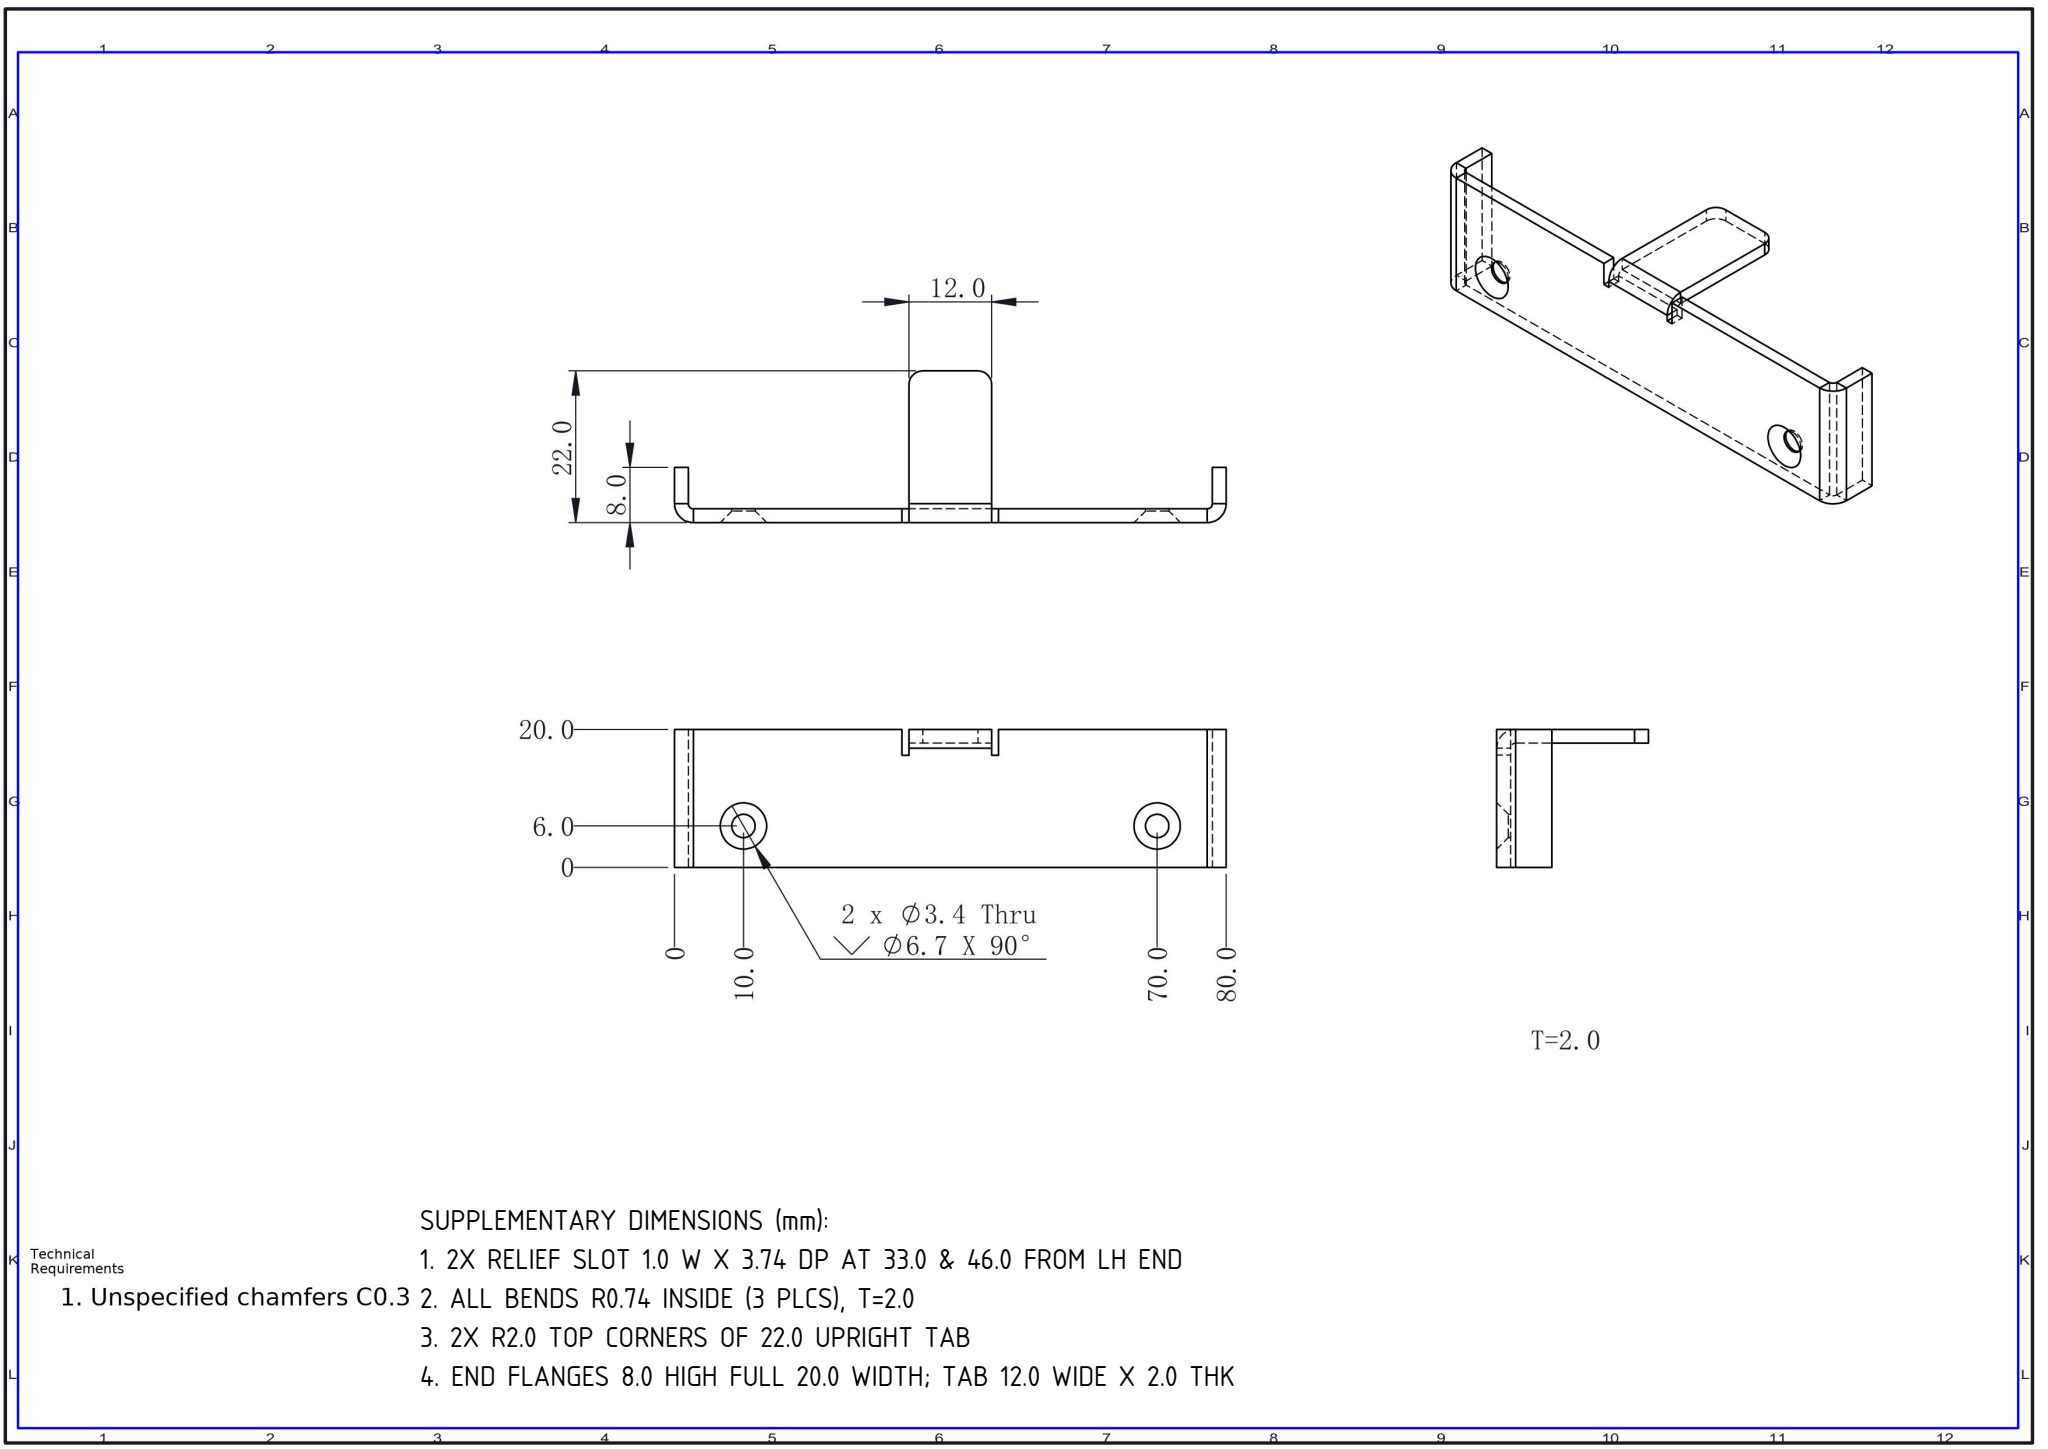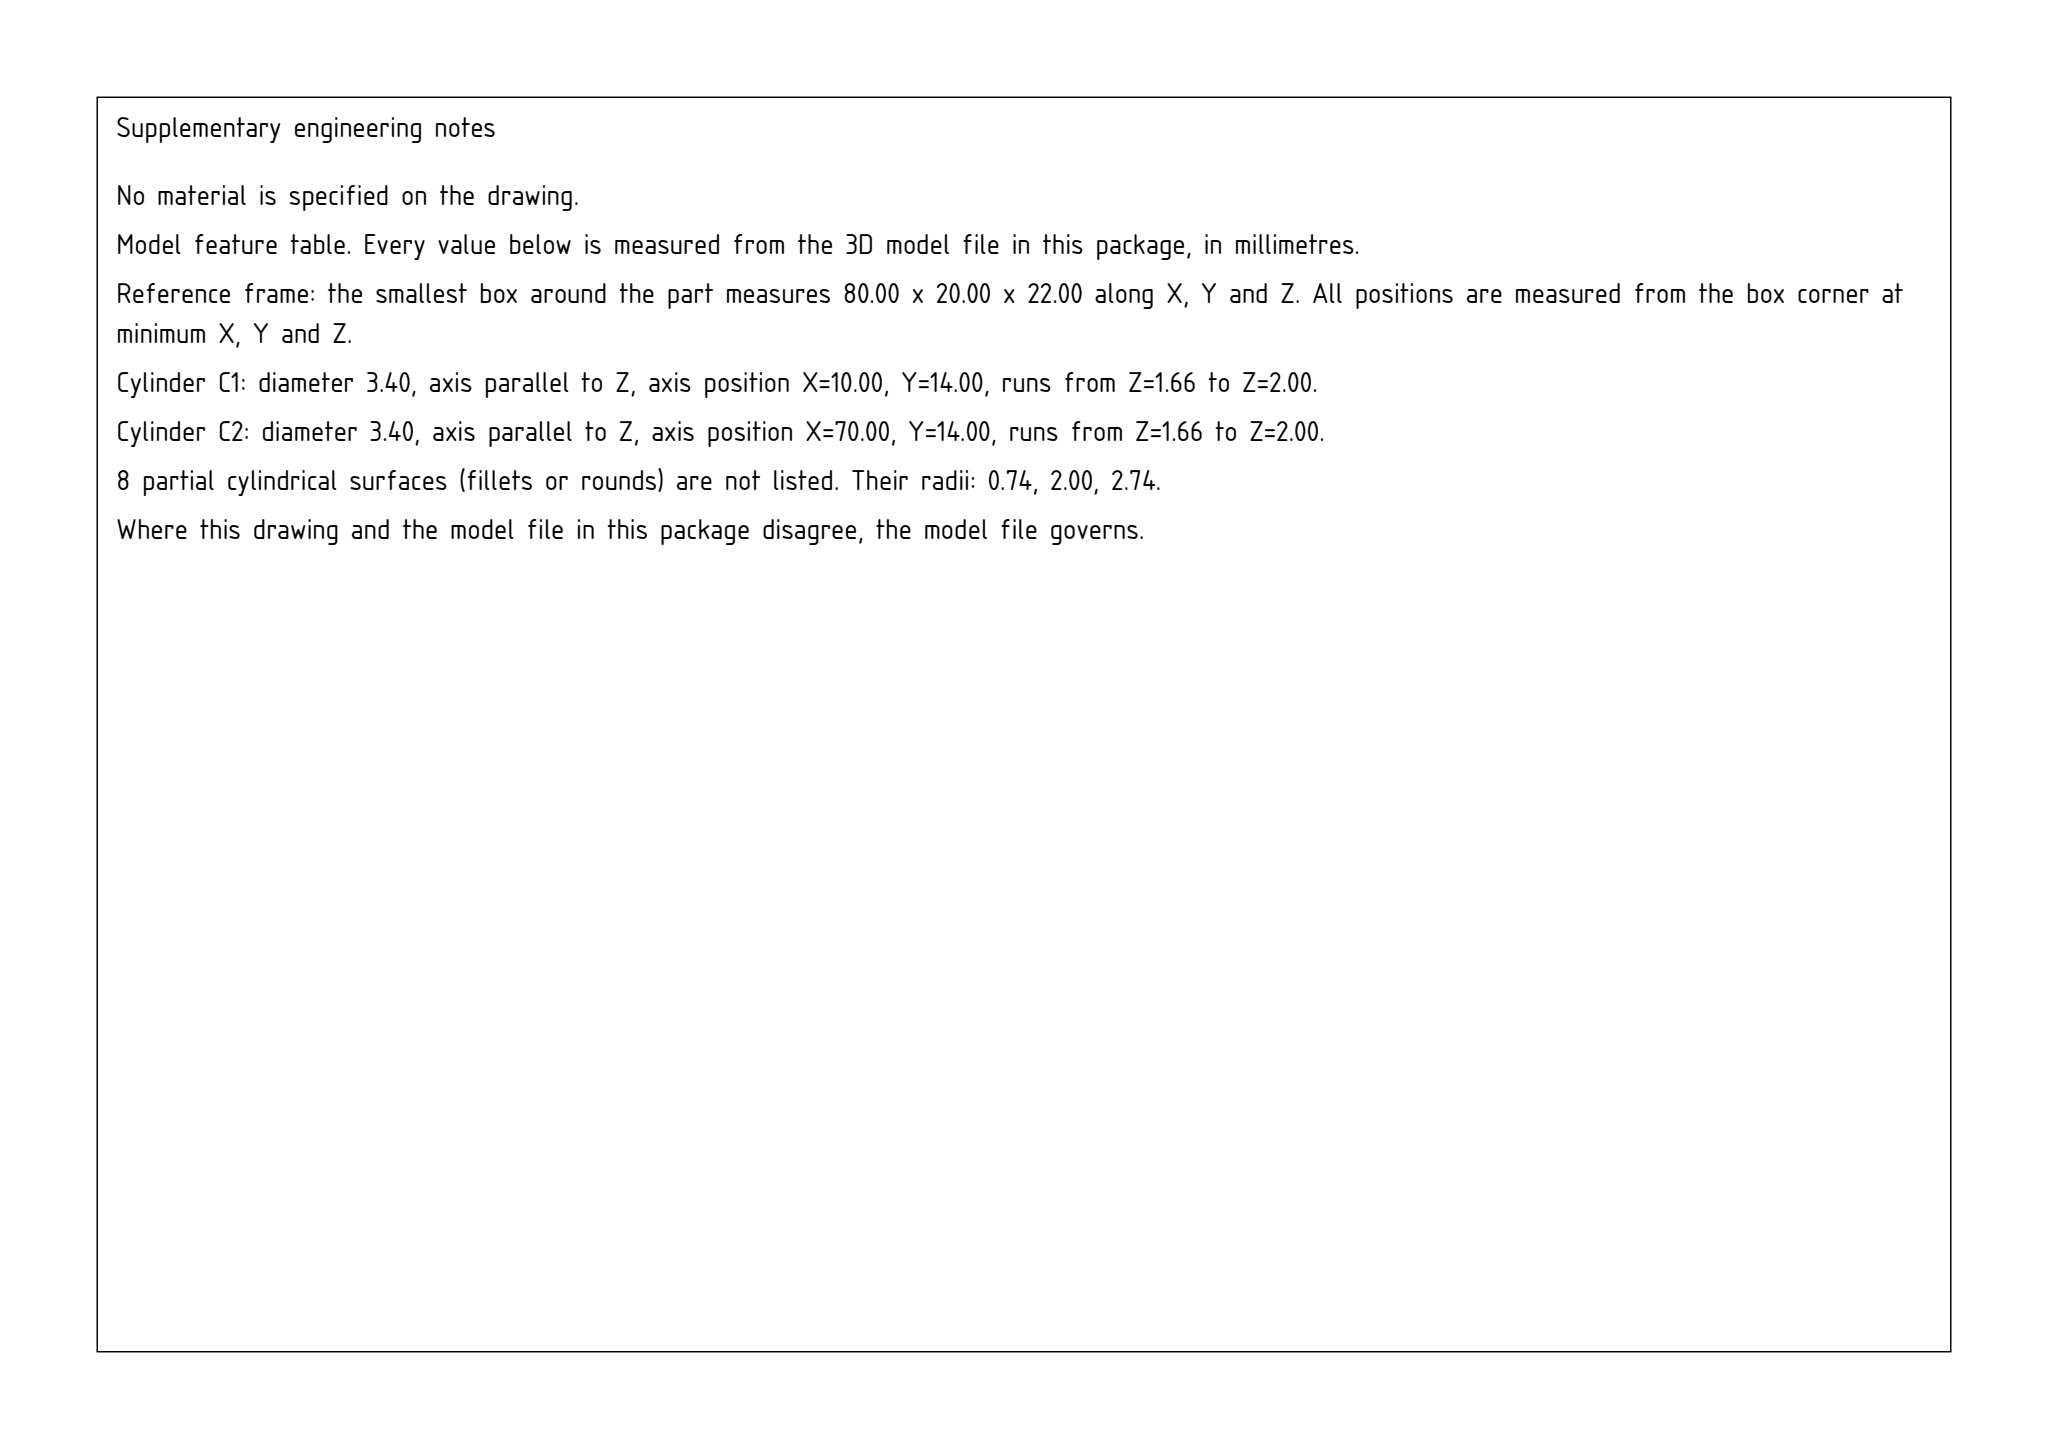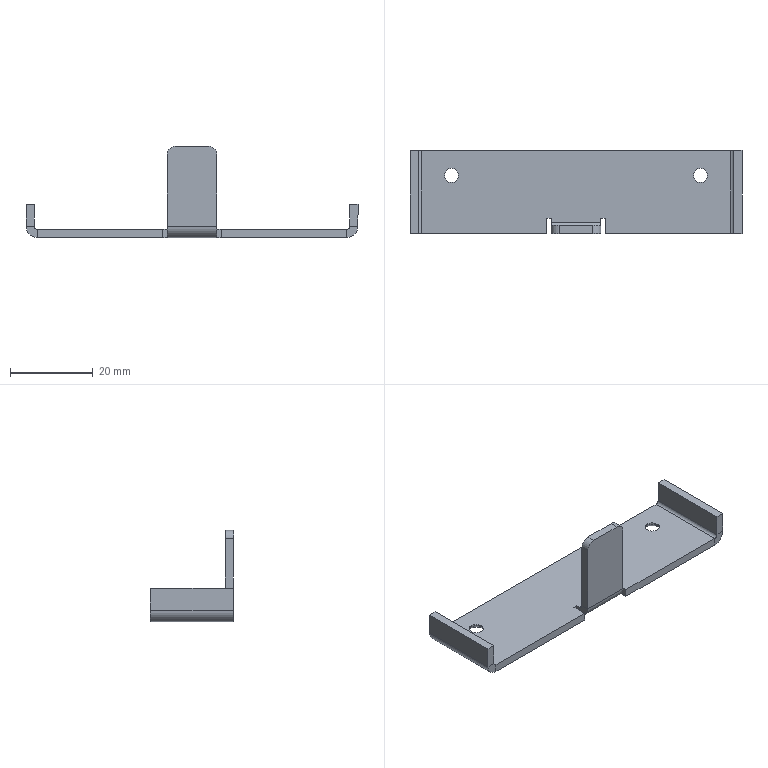Part | SolidWorks | mm | 1 solid | 48 faces | box 80 x 20 x 22 mm | volume 3989 mm3 | plane 32 | cylinder 12 | cone 4 | commonest cylinder face diameters 3.4 x4 5.473 x3 1.473 x3 4 x2